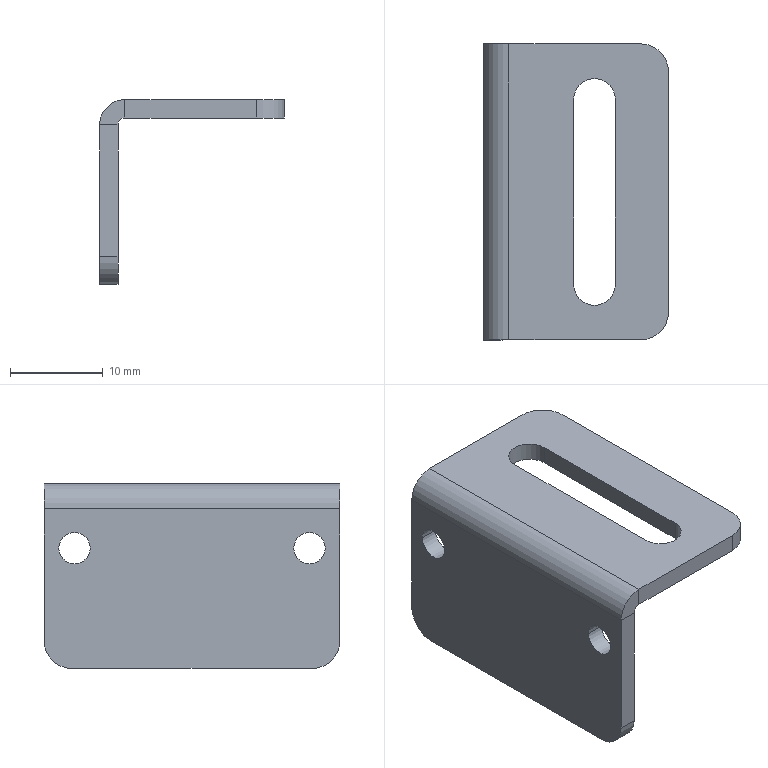Component | SolidWorks | 09-1111-12 | 1 solid | 26 faces | box 20 x 32 x 20 mm | volume 2121 mm3 | plane 14 | cylinder 12 | commonest cylinder face diameters 3.4 x4 6 x4 4.5 x2 5.473 x1 1.473 x1
STEP:
#1=COLOUR_RGB('',0.7922,0.8196,0.9333);
#2=FILL_AREA_STYLE_COLOUR('',#1);
#3=FILL_AREA_STYLE('',(#2));
#4=SURFACE_STYLE_FILL_AREA(#3);
#5=SURFACE_SIDE_STYLE('',(#4));
#6=SURFACE_STYLE_USAGE(.BOTH.,#5);
#7=PRESENTATION_STYLE_ASSIGNMENT((#6));
#8=CARTESIAN_POINT('',(5.115,16.78,49.727));
#9=VERTEX_POINT('',#8);
#10=CARTESIAN_POINT('',(5.115,16.914,49.727));
#11=VERTEX_POINT('',#10);
#12=CARTESIAN_POINT('',(5.115,16.847,49.727));
#13=DIRECTION('',(-1.,-0.,0.));
#14=DIRECTION('',(0.,1.,0.));
#15=AXIS2_PLACEMENT_3D('',#12,#13,#14);
#16=CIRCLE('',#15,0.06693);
#17=EDGE_CURVE('',#9,#11,#16,.T.);
#18=ORIENTED_EDGE('',*,*,#17,.F.);
#19=CARTESIAN_POINT('',(5.037,16.78,49.727));
#20=VERTEX_POINT('',#19);
#21=CARTESIAN_POINT('',(5.037,16.78,49.727));
#22=DIRECTION('',(-1.,-0.,0.));
#23=VECTOR('',#22,39.37);
#24=LINE('',#21,#23);
#25=EDGE_CURVE('',#9,#20,#24,.T.);
#26=ORIENTED_EDGE('',*,*,#25,.T.);
#27=CARTESIAN_POINT('',(5.037,16.914,49.727));
#28=VERTEX_POINT('',#27);
#29=CARTESIAN_POINT('',(5.037,16.847,49.727));
#30=DIRECTION('',(-1.,-0.,0.));
#31=DIRECTION('',(0.,1.,0.));
#32=AXIS2_PLACEMENT_3D('',#29,#30,#31);
#33=CIRCLE('',#32,0.06693);
#34=EDGE_CURVE('',#20,#28,#33,.T.);
#35=ORIENTED_EDGE('',*,*,#34,.T.);
#36=CARTESIAN_POINT('',(5.037,16.914,49.727));
#37=DIRECTION('',(-1.,-0.,0.));
#38=VECTOR('',#37,39.37);
#39=LINE('',#36,#38);
#40=EDGE_CURVE('',#11,#28,#39,.T.);
#41=ORIENTED_EDGE('',*,*,#40,.F.);
#42=EDGE_LOOP('',(#18,#26,#35,#41));
#43=FACE_OUTER_BOUND('',#42,.T.);
#44=CARTESIAN_POINT('',(5.037,16.847,49.727));
#45=DIRECTION('',(-1.,-0.,0.));
#46=DIRECTION('',(0.,1.,0.));
#47=AXIS2_PLACEMENT_3D('',#44,#45,#46);
#48=CYLINDRICAL_SURFACE('',#47,0.06693);
#49=ADVANCED_FACE('',(#43),#48,.F.);
#50=CARTESIAN_POINT('',(5.115,15.78,49.727));
#51=VERTEX_POINT('',#50);
#52=CARTESIAN_POINT('',(5.115,15.914,49.727));
#53=VERTEX_POINT('',#52);
#54=CARTESIAN_POINT('',(5.115,15.847,49.727));
#55=DIRECTION('',(-1.,-0.,0.));
#56=DIRECTION('',(0.,1.,0.));
#57=AXIS2_PLACEMENT_3D('',#54,#55,#56);
#58=CIRCLE('',#57,0.06693);
#59=EDGE_CURVE('',#51,#53,#58,.T.);
#60=ORIENTED_EDGE('',*,*,#59,.F.);
#61=CARTESIAN_POINT('',(5.037,15.78,49.727));
#62=VERTEX_POINT('',#61);
#63=CARTESIAN_POINT('',(5.037,15.78,49.727));
#64=DIRECTION('',(-1.,-0.,0.));
#65=VECTOR('',#64,39.37);
#66=LINE('',#63,#65);
#67=EDGE_CURVE('',#51,#62,#66,.T.);
#68=ORIENTED_EDGE('',*,*,#67,.T.);
#69=CARTESIAN_POINT('',(5.037,15.914,49.727));
#70=VERTEX_POINT('',#69);
#71=CARTESIAN_POINT('',(5.037,15.847,49.727));
#72=DIRECTION('',(-1.,-0.,0.));
#73=DIRECTION('',(0.,1.,0.));
#74=AXIS2_PLACEMENT_3D('',#71,#72,#73);
#75=CIRCLE('',#74,0.06693);
#76=EDGE_CURVE('',#62,#70,#75,.T.);
#77=ORIENTED_EDGE('',*,*,#76,.T.);
#78=CARTESIAN_POINT('',(5.037,15.914,49.727));
#79=DIRECTION('',(-1.,-0.,0.));
#80=VECTOR('',#79,39.37);
#81=LINE('',#78,#80);
#82=EDGE_CURVE('',#53,#70,#81,.T.);
#83=ORIENTED_EDGE('',*,*,#82,.F.);
#84=EDGE_LOOP('',(#60,#68,#77,#83));
#85=FACE_OUTER_BOUND('',#84,.T.);
#86=CARTESIAN_POINT('',(5.037,15.847,49.727));
#87=DIRECTION('',(-1.,-0.,0.));
#88=DIRECTION('',(0.,1.,0.));
#89=AXIS2_PLACEMENT_3D('',#86,#87,#88);
#90=CYLINDRICAL_SURFACE('',#89,0.06693);
#91=ADVANCED_FACE('',(#85),#90,.F.);
#92=CARTESIAN_POINT('',(5.037,16.977,49.894));
#93=VERTEX_POINT('',#92);
#94=CARTESIAN_POINT('',(5.115,16.977,49.894));
#95=VERTEX_POINT('',#94);
#96=CARTESIAN_POINT('',(5.037,16.977,49.894));
#97=DIRECTION('',(1.,0.,-0.));
#98=VECTOR('',#97,39.37);
#99=LINE('',#96,#98);
#100=EDGE_CURVE('',#93,#95,#99,.T.);
#101=ORIENTED_EDGE('',*,*,#100,.F.);
#102=CARTESIAN_POINT('',(5.144,16.977,50.002));
#103=VERTEX_POINT('',#102);
#104=CARTESIAN_POINT('',(5.144,16.977,49.894));
#105=DIRECTION('',(0.,-1.,0.));
#106=DIRECTION('',(1.,0.,0.));
#107=AXIS2_PLACEMENT_3D('',#104,#105,#106);
#108=CIRCLE('',#107,0.1077);
#109=EDGE_CURVE('',#103,#93,#108,.T.);
#110=ORIENTED_EDGE('',*,*,#109,.F.);
#111=CARTESIAN_POINT('',(5.144,16.977,49.923));
#112=VERTEX_POINT('',#111);
#113=CARTESIAN_POINT('',(5.144,16.977,49.923));
#114=DIRECTION('',(0.,0.,1.));
#115=VECTOR('',#114,39.37);
#116=LINE('',#113,#115);
#117=EDGE_CURVE('',#112,#103,#116,.T.);
#118=ORIENTED_EDGE('',*,*,#117,.F.);
#119=CARTESIAN_POINT('',(5.144,16.977,49.894));
#120=DIRECTION('',(0.,-1.,0.));
#121=DIRECTION('',(1.,0.,0.));
#122=AXIS2_PLACEMENT_3D('',#119,#120,#121);
#123=CIRCLE('',#122,0.029);
#124=EDGE_CURVE('',#112,#95,#123,.T.);
#125=ORIENTED_EDGE('',*,*,#124,.T.);
#126=EDGE_LOOP('',(#101,#110,#118,#125));
#127=FACE_OUTER_BOUND('',#126,.T.);
#128=CARTESIAN_POINT('',(5.037,16.977,49.894));
#129=DIRECTION('',(-0.,1.,-0.));
#130=DIRECTION('',(1.,0.,-0.));
#131=AXIS2_PLACEMENT_3D('',#128,#129,#130);
#132=PLANE('',#131);
#133=ADVANCED_FACE('',(#127),#132,.T.);
#134=CARTESIAN_POINT('',(5.115,16.977,49.333));
#135=VERTEX_POINT('',#134);
#136=CARTESIAN_POINT('',(5.115,16.977,50.002));
#137=DIRECTION('',(-0.,-0.,-1.));
#138=VECTOR('',#137,39.37);
#139=LINE('',#136,#138);
#140=EDGE_CURVE('',#95,#135,#139,.T.);
#141=ORIENTED_EDGE('',*,*,#140,.T.);
#142=CARTESIAN_POINT('',(5.037,16.977,49.333));
#143=VERTEX_POINT('',#142);
#144=CARTESIAN_POINT('',(5.144,16.977,49.333));
#145=DIRECTION('',(-1.,-0.,0.));
#146=VECTOR('',#145,39.37);
#147=LINE('',#144,#146);
#148=EDGE_CURVE('',#135,#143,#147,.T.);
#149=ORIENTED_EDGE('',*,*,#148,.T.);
#150=CARTESIAN_POINT('',(5.037,16.977,50.002));
#151=DIRECTION('',(-0.,-0.,-1.));
#152=VECTOR('',#151,39.37);
#153=LINE('',#150,#152);
#154=EDGE_CURVE('',#93,#143,#153,.T.);
#155=ORIENTED_EDGE('',*,*,#154,.F.);
#156=ORIENTED_EDGE('',*,*,#100,.T.);
#157=EDGE_LOOP('',(#141,#149,#155,#156));
#158=FACE_OUTER_BOUND('',#157,.T.);
#159=CARTESIAN_POINT('',(5.144,16.977,49.923));
#160=DIRECTION('',(-0.,1.,-0.));
#161=DIRECTION('',(1.,0.,-0.));
#162=AXIS2_PLACEMENT_3D('',#159,#160,#161);
#163=PLANE('',#162);
#164=ADVANCED_FACE('',(#158),#163,.T.);
#165=CARTESIAN_POINT('',(5.144,15.717,50.002));
#166=VERTEX_POINT('',#165);
#167=CARTESIAN_POINT('',(5.144,15.717,49.923));
#168=VERTEX_POINT('',#167);
#169=CARTESIAN_POINT('',(5.144,15.717,50.002));
#170=DIRECTION('',(-0.,-0.,-1.));
#171=VECTOR('',#170,39.37);
#172=LINE('',#169,#171);
#173=EDGE_CURVE('',#166,#168,#172,.T.);
#174=ORIENTED_EDGE('',*,*,#173,.F.);
#175=CARTESIAN_POINT('',(5.037,15.717,49.894));
#176=VERTEX_POINT('',#175);
#177=CARTESIAN_POINT('',(5.144,15.717,49.894));
#178=DIRECTION('',(0.,-1.,0.));
#179=DIRECTION('',(1.,0.,0.));
#180=AXIS2_PLACEMENT_3D('',#177,#178,#179);
#181=CIRCLE('',#180,0.1077);
#182=EDGE_CURVE('',#166,#176,#181,.T.);
#183=ORIENTED_EDGE('',*,*,#182,.T.);
#184=CARTESIAN_POINT('',(5.115,15.717,49.894));
#185=VERTEX_POINT('',#184);
#186=CARTESIAN_POINT('',(5.115,15.717,49.894));
#187=DIRECTION('',(-1.,-0.,0.));
#188=VECTOR('',#187,39.37);
#189=LINE('',#186,#188);
#190=EDGE_CURVE('',#185,#176,#189,.T.);
#191=ORIENTED_EDGE('',*,*,#190,.F.);
#192=CARTESIAN_POINT('',(5.144,15.717,49.894));
#193=DIRECTION('',(0.,-1.,0.));
#194=DIRECTION('',(1.,0.,0.));
#195=AXIS2_PLACEMENT_3D('',#192,#193,#194);
#196=CIRCLE('',#195,0.029);
#197=EDGE_CURVE('',#168,#185,#196,.T.);
#198=ORIENTED_EDGE('',*,*,#197,.F.);
#199=EDGE_LOOP('',(#174,#183,#191,#198));
#200=FACE_OUTER_BOUND('',#199,.T.);
#201=CARTESIAN_POINT('',(5.144,15.717,50.002));
#202=DIRECTION('',(0.,-1.,0.));
#203=DIRECTION('',(-1.,-0.,0.));
#204=AXIS2_PLACEMENT_3D('',#201,#202,#203);
#205=PLANE('',#204);
#206=ADVANCED_FACE('',(#200),#205,.T.);
#207=CARTESIAN_POINT('',(5.706,15.717,49.923));
#208=VERTEX_POINT('',#207);
#209=CARTESIAN_POINT('',(5.824,15.717,49.923));
#210=DIRECTION('',(-1.,-0.,0.));
#211=VECTOR('',#210,39.37);
#212=LINE('',#209,#211);
#213=EDGE_CURVE('',#208,#168,#212,.T.);
#214=ORIENTED_EDGE('',*,*,#213,.F.);
#215=CARTESIAN_POINT('',(5.706,15.717,50.002));
#216=VERTEX_POINT('',#215);
#217=CARTESIAN_POINT('',(5.706,15.717,49.894));
#218=DIRECTION('',(0.,0.,1.));
#219=VECTOR('',#218,39.37);
#220=LINE('',#217,#219);
#221=EDGE_CURVE('',#208,#216,#220,.T.);
#222=ORIENTED_EDGE('',*,*,#221,.T.);
#223=CARTESIAN_POINT('',(5.824,15.717,50.002));
#224=DIRECTION('',(-1.,-0.,0.));
#225=VECTOR('',#224,39.37);
#226=LINE('',#223,#225);
#227=EDGE_CURVE('',#216,#166,#226,.T.);
#228=ORIENTED_EDGE('',*,*,#227,.T.);
#229=ORIENTED_EDGE('',*,*,#173,.T.);
#230=EDGE_LOOP('',(#214,#222,#228,#229));
#231=FACE_OUTER_BOUND('',#230,.T.);
#232=CARTESIAN_POINT('',(5.115,15.717,49.894));
#233=DIRECTION('',(0.,-1.,0.));
#234=DIRECTION('',(-1.,-0.,0.));
#235=AXIS2_PLACEMENT_3D('',#232,#233,#234);
#236=PLANE('',#235);
#237=ADVANCED_FACE('',(#231),#236,.T.);
#238=CARTESIAN_POINT('',(5.115,16.847,49.727));
#239=DIRECTION('',(-1.,-0.,0.));
#240=DIRECTION('',(0.,1.,0.));
#241=AXIS2_PLACEMENT_3D('',#238,#239,#240);
#242=CIRCLE('',#241,0.06693);
#243=EDGE_CURVE('',#11,#9,#242,.T.);
#244=ORIENTED_EDGE('',*,*,#243,.T.);
#245=ORIENTED_EDGE('',*,*,#17,.T.);
#246=EDGE_LOOP('',(#244,#245));
#247=FACE_BOUND('',#246,.T.);
#248=CARTESIAN_POINT('',(5.115,15.847,49.727));
#249=DIRECTION('',(-1.,-0.,0.));
#250=DIRECTION('',(0.,1.,0.));
#251=AXIS2_PLACEMENT_3D('',#248,#249,#250);
#252=CIRCLE('',#251,0.06693);
#253=EDGE_CURVE('',#53,#51,#252,.T.);
#254=ORIENTED_EDGE('',*,*,#253,.T.);
#255=ORIENTED_EDGE('',*,*,#59,.T.);
#256=EDGE_LOOP('',(#254,#255));
#257=FACE_BOUND('',#256,.T.);
#258=CARTESIAN_POINT('',(5.115,16.859,49.215));
#259=VERTEX_POINT('',#258);
#260=CARTESIAN_POINT('',(5.115,15.836,49.215));
#261=VERTEX_POINT('',#260);
#262=CARTESIAN_POINT('',(5.115,16.977,49.215));
#263=DIRECTION('',(0.,-1.,0.));
#264=VECTOR('',#263,39.37);
#265=LINE('',#262,#264);
#266=EDGE_CURVE('',#259,#261,#265,.T.);
#267=ORIENTED_EDGE('',*,*,#266,.F.);
#268=CARTESIAN_POINT('',(5.115,16.859,49.333));
#269=DIRECTION('',(1.,0.,-0.));
#270=DIRECTION('',(0.,1.,0.));
#271=AXIS2_PLACEMENT_3D('',#268,#269,#270);
#272=CIRCLE('',#271,0.1181);
#273=EDGE_CURVE('',#259,#135,#272,.T.);
#274=ORIENTED_EDGE('',*,*,#273,.T.);
#275=ORIENTED_EDGE('',*,*,#140,.F.);
#276=CARTESIAN_POINT('',(5.115,16.977,49.894));
#277=DIRECTION('',(0.,-1.,0.));
#278=VECTOR('',#277,39.37);
#279=LINE('',#276,#278);
#280=EDGE_CURVE('',#95,#185,#279,.T.);
#281=ORIENTED_EDGE('',*,*,#280,.T.);
#282=CARTESIAN_POINT('',(5.115,15.717,49.333));
#283=VERTEX_POINT('',#282);
#284=CARTESIAN_POINT('',(5.115,15.717,50.002));
#285=DIRECTION('',(-0.,-0.,-1.));
#286=VECTOR('',#285,39.37);
#287=LINE('',#284,#286);
#288=EDGE_CURVE('',#185,#283,#287,.T.);
#289=ORIENTED_EDGE('',*,*,#288,.T.);
#290=CARTESIAN_POINT('',(5.115,15.836,49.333));
#291=DIRECTION('',(1.,0.,-0.));
#292=DIRECTION('',(0.,1.,0.));
#293=AXIS2_PLACEMENT_3D('',#290,#291,#292);
#294=CIRCLE('',#293,0.1181);
#295=EDGE_CURVE('',#283,#261,#294,.T.);
#296=ORIENTED_EDGE('',*,*,#295,.T.);
#297=EDGE_LOOP('',(#267,#274,#275,#281,#289,#296));
#298=FACE_OUTER_BOUND('',#297,.T.);
#299=CARTESIAN_POINT('',(5.115,16.977,50.002));
#300=DIRECTION('',(-1.,-0.,0.));
#301=DIRECTION('',(-0.,1.,-0.));
#302=AXIS2_PLACEMENT_3D('',#299,#300,#301);
#303=PLANE('',#302);
#304=ADVANCED_FACE('',(#247,#257,#298),#303,.F.);
#305=CARTESIAN_POINT('',(5.037,16.859,49.215));
#306=VERTEX_POINT('',#305);
#307=CARTESIAN_POINT('',(5.037,15.836,49.215));
#308=VERTEX_POINT('',#307);
#309=CARTESIAN_POINT('',(5.037,16.977,49.215));
#310=DIRECTION('',(0.,-1.,0.));
#311=VECTOR('',#310,39.37);
#312=LINE('',#309,#311);
#313=EDGE_CURVE('',#306,#308,#312,.T.);
#314=ORIENTED_EDGE('',*,*,#313,.F.);
#315=CARTESIAN_POINT('',(5.037,16.859,49.215));
#316=DIRECTION('',(1.,0.,-0.));
#317=VECTOR('',#316,39.37);
#318=LINE('',#315,#317);
#319=EDGE_CURVE('',#306,#259,#318,.T.);
#320=ORIENTED_EDGE('',*,*,#319,.T.);
#321=ORIENTED_EDGE('',*,*,#266,.T.);
#322=CARTESIAN_POINT('',(5.037,15.836,49.215));
#323=DIRECTION('',(-1.,-0.,0.));
#324=VECTOR('',#323,39.37);
#325=LINE('',#322,#324);
#326=EDGE_CURVE('',#261,#308,#325,.T.);
#327=ORIENTED_EDGE('',*,*,#326,.T.);
#328=EDGE_LOOP('',(#314,#320,#321,#327));
#329=FACE_OUTER_BOUND('',#328,.T.);
#330=CARTESIAN_POINT('',(5.037,16.977,49.215));
#331=DIRECTION('',(-0.,-0.,-1.));
#332=DIRECTION('',(-0.,1.,-0.));
#333=AXIS2_PLACEMENT_3D('',#330,#331,#332);
#334=PLANE('',#333);
#335=ADVANCED_FACE('',(#329),#334,.T.);
#336=CARTESIAN_POINT('',(5.037,16.847,49.727));
#337=DIRECTION('',(-1.,-0.,0.));
#338=DIRECTION('',(0.,1.,0.));
#339=AXIS2_PLACEMENT_3D('',#336,#337,#338);
#340=CIRCLE('',#339,0.06693);
#341=EDGE_CURVE('',#28,#20,#340,.T.);
#342=ORIENTED_EDGE('',*,*,#341,.F.);
#343=ORIENTED_EDGE('',*,*,#34,.F.);
#344=EDGE_LOOP('',(#342,#343));
#345=FACE_BOUND('',#344,.T.);
#346=CARTESIAN_POINT('',(5.037,15.847,49.727));
#347=DIRECTION('',(-1.,-0.,0.));
#348=DIRECTION('',(0.,1.,0.));
#349=AXIS2_PLACEMENT_3D('',#346,#347,#348);
#350=CIRCLE('',#349,0.06693);
#351=EDGE_CURVE('',#70,#62,#350,.T.);
#352=ORIENTED_EDGE('',*,*,#351,.F.);
#353=ORIENTED_EDGE('',*,*,#76,.F.);
#354=EDGE_LOOP('',(#352,#353));
#355=FACE_BOUND('',#354,.T.);
#356=ORIENTED_EDGE('',*,*,#154,.T.);
#357=CARTESIAN_POINT('',(5.037,16.859,49.333));
#358=DIRECTION('',(-1.,-0.,0.));
#359=DIRECTION('',(0.,1.,0.));
#360=AXIS2_PLACEMENT_3D('',#357,#358,#359);
#361=CIRCLE('',#360,0.1181);
#362=EDGE_CURVE('',#143,#306,#361,.T.);
#363=ORIENTED_EDGE('',*,*,#362,.T.);
#364=ORIENTED_EDGE('',*,*,#313,.T.);
#365=CARTESIAN_POINT('',(5.037,15.717,49.333));
#366=VERTEX_POINT('',#365);
#367=CARTESIAN_POINT('',(5.037,15.836,49.333));
#368=DIRECTION('',(-1.,-0.,0.));
#369=DIRECTION('',(0.,1.,0.));
#370=AXIS2_PLACEMENT_3D('',#367,#368,#369);
#371=CIRCLE('',#370,0.1181);
#372=EDGE_CURVE('',#308,#366,#371,.T.);
#373=ORIENTED_EDGE('',*,*,#372,.T.);
#374=CARTESIAN_POINT('',(5.037,15.717,50.002));
#375=DIRECTION('',(-0.,-0.,-1.));
#376=VECTOR('',#375,39.37);
#377=LINE('',#374,#376);
#378=EDGE_CURVE('',#176,#366,#377,.T.);
#379=ORIENTED_EDGE('',*,*,#378,.F.);
#380=CARTESIAN_POINT('',(5.037,16.977,49.894));
#381=DIRECTION('',(0.,-1.,0.));
#382=VECTOR('',#381,39.37);
#383=LINE('',#380,#382);
#384=EDGE_CURVE('',#93,#176,#383,.T.);
#385=ORIENTED_EDGE('',*,*,#384,.F.);
#386=EDGE_LOOP('',(#356,#363,#364,#373,#379,#385));
#387=FACE_OUTER_BOUND('',#386,.T.);
#388=CARTESIAN_POINT('',(5.037,16.977,50.002));
#389=DIRECTION('',(-1.,-0.,0.));
#390=DIRECTION('',(-0.,1.,-0.));
#391=AXIS2_PLACEMENT_3D('',#388,#389,#390);
#392=PLANE('',#391);
#393=ADVANCED_FACE('',(#345,#355,#387),#392,.T.);
#394=ORIENTED_EDGE('',*,*,#182,.F.);
#395=CARTESIAN_POINT('',(5.144,16.977,50.002));
#396=DIRECTION('',(0.,-1.,0.));
#397=VECTOR('',#396,39.37);
#398=LINE('',#395,#397);
#399=EDGE_CURVE('',#103,#166,#398,.T.);
#400=ORIENTED_EDGE('',*,*,#399,.F.);
#401=ORIENTED_EDGE('',*,*,#109,.T.);
#402=ORIENTED_EDGE('',*,*,#384,.T.);
#403=EDGE_LOOP('',(#394,#400,#401,#402));
#404=FACE_OUTER_BOUND('',#403,.T.);
#405=CARTESIAN_POINT('',(5.144,16.977,49.894));
#406=DIRECTION('',(0.,-1.,0.));
#407=DIRECTION('',(-1.,0.,0.));
#408=AXIS2_PLACEMENT_3D('',#405,#406,#407);
#409=CYLINDRICAL_SURFACE('',#408,0.1077);
#410=ADVANCED_FACE('',(#404),#409,.T.);
#411=CARTESIAN_POINT('',(5.42,16.741,50.002));
#412=VERTEX_POINT('',#411);
#413=CARTESIAN_POINT('',(5.598,16.741,50.002));
#414=VERTEX_POINT('',#413);
#415=CARTESIAN_POINT('',(5.509,16.741,50.002));
#416=DIRECTION('',(-0.,-0.,-1.));
#417=DIRECTION('',(-1.,0.,0.));
#418=AXIS2_PLACEMENT_3D('',#415,#416,#417);
#419=CIRCLE('',#418,0.08858);
#420=EDGE_CURVE('',#412,#414,#419,.T.);
#421=ORIENTED_EDGE('',*,*,#420,.T.);
#422=CARTESIAN_POINT('',(5.598,15.954,50.002));
#423=VERTEX_POINT('',#422);
#424=CARTESIAN_POINT('',(5.598,16.741,50.002));
#425=DIRECTION('',(0.,-1.,0.));
#426=VECTOR('',#425,39.37);
#427=LINE('',#424,#426);
#428=EDGE_CURVE('',#414,#423,#427,.T.);
#429=ORIENTED_EDGE('',*,*,#428,.T.);
#430=CARTESIAN_POINT('',(5.42,15.954,50.002));
#431=VERTEX_POINT('',#430);
#432=CARTESIAN_POINT('',(5.509,15.954,50.002));
#433=DIRECTION('',(-0.,-0.,-1.));
#434=DIRECTION('',(-1.,0.,0.));
#435=AXIS2_PLACEMENT_3D('',#432,#433,#434);
#436=CIRCLE('',#435,0.08858);
#437=EDGE_CURVE('',#423,#431,#436,.T.);
#438=ORIENTED_EDGE('',*,*,#437,.T.);
#439=CARTESIAN_POINT('',(5.42,16.741,50.002));
#440=DIRECTION('',(-0.,1.,-0.));
#441=VECTOR('',#440,39.37);
#442=LINE('',#439,#441);
#443=EDGE_CURVE('',#431,#412,#442,.T.);
#444=ORIENTED_EDGE('',*,*,#443,.T.);
#445=EDGE_LOOP('',(#421,#429,#438,#444));
#446=FACE_BOUND('',#445,.T.);
#447=ORIENTED_EDGE('',*,*,#227,.F.);
#448=CARTESIAN_POINT('',(5.824,15.836,50.002));
#449=VERTEX_POINT('',#448);
#450=CARTESIAN_POINT('',(5.706,15.836,50.002));
#451=DIRECTION('',(0.,0.,1.));
#452=DIRECTION('',(1.,0.,0.));
#453=AXIS2_PLACEMENT_3D('',#450,#451,#452);
#454=CIRCLE('',#453,0.1181);
#455=EDGE_CURVE('',#216,#449,#454,.T.);
#456=ORIENTED_EDGE('',*,*,#455,.T.);
#457=CARTESIAN_POINT('',(5.824,16.859,50.002));
#458=VERTEX_POINT('',#457);
#459=CARTESIAN_POINT('',(5.824,16.977,50.002));
#460=DIRECTION('',(0.,-1.,0.));
#461=VECTOR('',#460,39.37);
#462=LINE('',#459,#461);
#463=EDGE_CURVE('',#458,#449,#462,.T.);
#464=ORIENTED_EDGE('',*,*,#463,.F.);
#465=CARTESIAN_POINT('',(5.706,16.977,50.002));
#466=VERTEX_POINT('',#465);
#467=CARTESIAN_POINT('',(5.706,16.859,50.002));
#468=DIRECTION('',(0.,0.,1.));
#469=DIRECTION('',(1.,0.,0.));
#470=AXIS2_PLACEMENT_3D('',#467,#468,#469);
#471=CIRCLE('',#470,0.1181);
#472=EDGE_CURVE('',#458,#466,#471,.T.);
#473=ORIENTED_EDGE('',*,*,#472,.T.);
#474=CARTESIAN_POINT('',(5.824,16.977,50.002));
#475=DIRECTION('',(-1.,-0.,0.));
#476=VECTOR('',#475,39.37);
#477=LINE('',#474,#476);
#478=EDGE_CURVE('',#466,#103,#477,.T.);
#479=ORIENTED_EDGE('',*,*,#478,.T.);
#480=ORIENTED_EDGE('',*,*,#399,.T.);
#481=EDGE_LOOP('',(#447,#456,#464,#473,#479,#480));
#482=FACE_OUTER_BOUND('',#481,.T.);
#483=CARTESIAN_POINT('',(5.824,16.977,50.002));
#484=DIRECTION('',(0.,0.,1.));
#485=DIRECTION('',(1.,0.,-0.));
#486=AXIS2_PLACEMENT_3D('',#483,#484,#485);
#487=PLANE('',#486);
#488=ADVANCED_FACE('',(#446,#482),#487,.T.);
#489=ORIENTED_EDGE('',*,*,#463,.T.);
#490=CARTESIAN_POINT('',(5.824,15.836,49.923));
#491=VERTEX_POINT('',#490);
#492=CARTESIAN_POINT('',(5.824,15.836,49.923));
#493=DIRECTION('',(-0.,-0.,-1.));
#494=VECTOR('',#493,39.37);
#495=LINE('',#492,#494);
#496=EDGE_CURVE('',#449,#491,#495,.T.);
#497=ORIENTED_EDGE('',*,*,#496,.T.);
#498=CARTESIAN_POINT('',(5.824,16.859,49.923));
#499=VERTEX_POINT('',#498);
#500=CARTESIAN_POINT('',(5.824,16.977,49.923));
#501=DIRECTION('',(0.,-1.,0.));
#502=VECTOR('',#501,39.37);
#503=LINE('',#500,#502);
#504=EDGE_CURVE('',#499,#491,#503,.T.);
#505=ORIENTED_EDGE('',*,*,#504,.F.);
#506=CARTESIAN_POINT('',(5.824,16.859,49.923));
#507=DIRECTION('',(0.,0.,1.));
#508=VECTOR('',#507,39.37);
#509=LINE('',#506,#508);
#510=EDGE_CURVE('',#499,#458,#509,.T.);
#511=ORIENTED_EDGE('',*,*,#510,.T.);
#512=EDGE_LOOP('',(#489,#497,#505,#511));
#513=FACE_OUTER_BOUND('',#512,.T.);
#514=CARTESIAN_POINT('',(5.824,16.977,49.923));
#515=DIRECTION('',(1.,0.,-0.));
#516=DIRECTION('',(-0.,-0.,-1.));
#517=AXIS2_PLACEMENT_3D('',#514,#515,#516);
#518=PLANE('',#517);
#519=ADVANCED_FACE('',(#513),#518,.T.);
#520=CARTESIAN_POINT('',(5.598,16.741,49.923));
#521=VERTEX_POINT('',#520);
#522=CARTESIAN_POINT('',(5.598,15.954,49.923));
#523=VERTEX_POINT('',#522);
#524=CARTESIAN_POINT('',(5.598,16.741,49.923));
#525=DIRECTION('',(0.,-1.,0.));
#526=VECTOR('',#525,39.37);
#527=LINE('',#524,#526);
#528=EDGE_CURVE('',#521,#523,#527,.T.);
#529=ORIENTED_EDGE('',*,*,#528,.F.);
#530=CARTESIAN_POINT('',(5.42,16.741,49.923));
#531=VERTEX_POINT('',#530);
#532=CARTESIAN_POINT('',(5.509,16.741,49.923));
#533=DIRECTION('',(-0.,-0.,-1.));
#534=DIRECTION('',(-1.,0.,0.));
#535=AXIS2_PLACEMENT_3D('',#532,#533,#534);
#536=CIRCLE('',#535,0.08858);
#537=EDGE_CURVE('',#531,#521,#536,.T.);
#538=ORIENTED_EDGE('',*,*,#537,.F.);
#539=CARTESIAN_POINT('',(5.42,15.954,49.923));
#540=VERTEX_POINT('',#539);
#541=CARTESIAN_POINT('',(5.42,16.741,49.923));
#542=DIRECTION('',(-0.,1.,-0.));
#543=VECTOR('',#542,39.37);
#544=LINE('',#541,#543);
#545=EDGE_CURVE('',#540,#531,#544,.T.);
#546=ORIENTED_EDGE('',*,*,#545,.F.);
#547=CARTESIAN_POINT('',(5.509,15.954,49.923));
#548=DIRECTION('',(-0.,-0.,-1.));
#549=DIRECTION('',(-1.,0.,0.));
#550=AXIS2_PLACEMENT_3D('',#547,#548,#549);
#551=CIRCLE('',#550,0.08858);
#552=EDGE_CURVE('',#523,#540,#551,.T.);
#553=ORIENTED_EDGE('',*,*,#552,.F.);
#554=EDGE_LOOP('',(#529,#538,#546,#553));
#555=FACE_BOUND('',#554,.T.);
#556=ORIENTED_EDGE('',*,*,#504,.T.);
#557=CARTESIAN_POINT('',(5.706,15.836,49.923));
#558=DIRECTION('',(-0.,-0.,-1.));
#559=DIRECTION('',(1.,0.,0.));
#560=AXIS2_PLACEMENT_3D('',#557,#558,#559);
#561=CIRCLE('',#560,0.1181);
#562=EDGE_CURVE('',#491,#208,#561,.T.);
#563=ORIENTED_EDGE('',*,*,#562,.T.);
#564=ORIENTED_EDGE('',*,*,#213,.T.);
#565=CARTESIAN_POINT('',(5.144,16.977,49.923));
#566=DIRECTION('',(0.,-1.,0.));
#567=VECTOR('',#566,39.37);
#568=LINE('',#565,#567);
#569=EDGE_CURVE('',#112,#168,#568,.T.);
#570=ORIENTED_EDGE('',*,*,#569,.F.);
#571=CARTESIAN_POINT('',(5.706,16.977,49.923));
#572=VERTEX_POINT('',#571);
#573=CARTESIAN_POINT('',(5.824,16.977,49.923));
#574=DIRECTION('',(-1.,-0.,0.));
#575=VECTOR('',#574,39.37);
#576=LINE('',#573,#575);
#577=EDGE_CURVE('',#572,#112,#576,.T.);
#578=ORIENTED_EDGE('',*,*,#577,.F.);
#579=CARTESIAN_POINT('',(5.706,16.859,49.923));
#580=DIRECTION('',(-0.,-0.,-1.));
#581=DIRECTION('',(1.,0.,0.));
#582=AXIS2_PLACEMENT_3D('',#579,#580,#581);
#583=CIRCLE('',#582,0.1181);
#584=EDGE_CURVE('',#572,#499,#583,.T.);
#585=ORIENTED_EDGE('',*,*,#584,.T.);
#586=EDGE_LOOP('',(#556,#563,#564,#570,#578,#585));
#587=FACE_OUTER_BOUND('',#586,.T.);
#588=CARTESIAN_POINT('',(5.824,16.977,49.923));
#589=DIRECTION('',(0.,0.,1.));
#590=DIRECTION('',(1.,0.,-0.));
#591=AXIS2_PLACEMENT_3D('',#588,#589,#590);
#592=PLANE('',#591);
#593=ADVANCED_FACE('',(#555,#587),#592,.F.);
#594=ORIENTED_EDGE('',*,*,#197,.T.);
#595=ORIENTED_EDGE('',*,*,#280,.F.);
#596=ORIENTED_EDGE('',*,*,#124,.F.);
#597=ORIENTED_EDGE('',*,*,#569,.T.);
#598=EDGE_LOOP('',(#594,#595,#596,#597));
#599=FACE_OUTER_BOUND('',#598,.T.);
#600=CARTESIAN_POINT('',(5.144,16.977,49.894));
#601=DIRECTION('',(0.,-1.,0.));
#602=DIRECTION('',(-1.,0.,0.));
#603=AXIS2_PLACEMENT_3D('',#600,#601,#602);
#604=CYLINDRICAL_SURFACE('',#603,0.029);
#605=ADVANCED_FACE('',(#599),#604,.F.);
#606=ORIENTED_EDGE('',*,*,#478,.F.);
#607=CARTESIAN_POINT('',(5.706,16.977,49.894));
#608=DIRECTION('',(-0.,-0.,-1.));
#609=VECTOR('',#608,39.37);
#610=LINE('',#607,#609);
#611=EDGE_CURVE('',#466,#572,#610,.T.);
#612=ORIENTED_EDGE('',*,*,#611,.T.);
#613=ORIENTED_EDGE('',*,*,#577,.T.);
#614=ORIENTED_EDGE('',*,*,#117,.T.);
#615=EDGE_LOOP('',(#606,#612,#613,#614));
#616=FACE_OUTER_BOUND('',#615,.T.);
#617=CARTESIAN_POINT('',(5.144,16.977,49.894));
#618=DIRECTION('',(-0.,1.,-0.));
#619=DIRECTION('',(1.,0.,-0.));
#620=AXIS2_PLACEMENT_3D('',#617,#618,#619);
#621=PLANE('',#620);
#622=ADVANCED_FACE('',(#616),#621,.T.);
#623=ORIENTED_EDGE('',*,*,#378,.T.);
#624=CARTESIAN_POINT('',(5.115,15.717,49.333));
#625=DIRECTION('',(1.,0.,-0.));
#626=VECTOR('',#625,39.37);
#627=LINE('',#624,#626);
#628=EDGE_CURVE('',#366,#283,#627,.T.);
#629=ORIENTED_EDGE('',*,*,#628,.T.);
#630=ORIENTED_EDGE('',*,*,#288,.F.);
#631=ORIENTED_EDGE('',*,*,#190,.T.);
#632=EDGE_LOOP('',(#623,#629,#630,#631));
#633=FACE_OUTER_BOUND('',#632,.T.);
#634=CARTESIAN_POINT('',(5.144,15.717,49.894));
#635=DIRECTION('',(-0.,1.,-0.));
#636=DIRECTION('',(1.,0.,-0.));
#637=AXIS2_PLACEMENT_3D('',#634,#635,#636);
#638=PLANE('',#637);
#639=ADVANCED_FACE('',(#633),#638,.F.);
#640=ORIENTED_EDGE('',*,*,#67,.F.);
#641=ORIENTED_EDGE('',*,*,#253,.F.);
#642=ORIENTED_EDGE('',*,*,#82,.T.);
#643=ORIENTED_EDGE('',*,*,#351,.T.);
#644=EDGE_LOOP('',(#640,#641,#642,#643));
#645=FACE_OUTER_BOUND('',#644,.T.);
#646=CARTESIAN_POINT('',(5.037,15.847,49.727));
#647=DIRECTION('',(-1.,-0.,0.));
#648=DIRECTION('',(0.,1.,0.));
#649=AXIS2_PLACEMENT_3D('',#646,#647,#648);
#650=CYLINDRICAL_SURFACE('',#649,0.06693);
#651=ADVANCED_FACE('',(#645),#650,.F.);
#652=ORIENTED_EDGE('',*,*,#25,.F.);
#653=ORIENTED_EDGE('',*,*,#243,.F.);
#654=ORIENTED_EDGE('',*,*,#40,.T.);
#655=ORIENTED_EDGE('',*,*,#341,.T.);
#656=EDGE_LOOP('',(#652,#653,#654,#655));
#657=FACE_OUTER_BOUND('',#656,.T.);
#658=CARTESIAN_POINT('',(5.037,16.847,49.727));
#659=DIRECTION('',(-1.,-0.,0.));
#660=DIRECTION('',(0.,1.,0.));
#661=AXIS2_PLACEMENT_3D('',#658,#659,#660);
#662=CYLINDRICAL_SURFACE('',#661,0.06693);
#663=ADVANCED_FACE('',(#657),#662,.F.);
#664=ORIENTED_EDGE('',*,*,#537,.T.);
#665=CARTESIAN_POINT('',(5.598,16.741,50.002));
#666=DIRECTION('',(-0.,-0.,-1.));
#667=VECTOR('',#666,39.37);
#668=LINE('',#665,#667);
#669=EDGE_CURVE('',#414,#521,#668,.T.);
#670=ORIENTED_EDGE('',*,*,#669,.F.);
#671=ORIENTED_EDGE('',*,*,#420,.F.);
#672=CARTESIAN_POINT('',(5.42,16.741,50.002));
#673=DIRECTION('',(-0.,-0.,-1.));
#674=VECTOR('',#673,39.37);
#675=LINE('',#672,#674);
#676=EDGE_CURVE('',#412,#531,#675,.T.);
#677=ORIENTED_EDGE('',*,*,#676,.T.);
#678=EDGE_LOOP('',(#664,#670,#671,#677));
#679=FACE_OUTER_BOUND('',#678,.T.);
#680=CARTESIAN_POINT('',(5.509,16.741,50.002));
#681=DIRECTION('',(-0.,-0.,-1.));
#682=DIRECTION('',(-1.,0.,0.));
#683=AXIS2_PLACEMENT_3D('',#680,#681,#682);
#684=CYLINDRICAL_SURFACE('',#683,0.08858);
#685=ADVANCED_FACE('',(#679),#684,.F.);
#686=ORIENTED_EDGE('',*,*,#545,.T.);
#687=ORIENTED_EDGE('',*,*,#676,.F.);
#688=ORIENTED_EDGE('',*,*,#443,.F.);
#689=CARTESIAN_POINT('',(5.42,15.954,50.002));
#690=DIRECTION('',(-0.,-0.,-1.));
#691=VECTOR('',#690,39.37);
#692=LINE('',#689,#691);
#693=EDGE_CURVE('',#431,#540,#692,.T.);
#694=ORIENTED_EDGE('',*,*,#693,.T.);
#695=EDGE_LOOP('',(#686,#687,#688,#694));
#696=FACE_OUTER_BOUND('',#695,.T.);
#697=CARTESIAN_POINT('',(5.42,16.741,50.002));
#698=DIRECTION('',(-1.,-0.,0.));
#699=DIRECTION('',(0.,0.,1.));
#700=AXIS2_PLACEMENT_3D('',#697,#698,#699);
#701=PLANE('',#700);
#702=ADVANCED_FACE('',(#696),#701,.F.);
#703=ORIENTED_EDGE('',*,*,#552,.T.);
#704=ORIENTED_EDGE('',*,*,#693,.F.);
#705=ORIENTED_EDGE('',*,*,#437,.F.);
#706=CARTESIAN_POINT('',(5.598,15.954,50.002));
#707=DIRECTION('',(-0.,-0.,-1.));
#708=VECTOR('',#707,39.37);
#709=LINE('',#706,#708);
#710=EDGE_CURVE('',#423,#523,#709,.T.);
#711=ORIENTED_EDGE('',*,*,#710,.T.);
#712=EDGE_LOOP('',(#703,#704,#705,#711));
#713=FACE_OUTER_BOUND('',#712,.T.);
#714=CARTESIAN_POINT('',(5.509,15.954,50.002));
#715=DIRECTION('',(-0.,-0.,-1.));
#716=DIRECTION('',(-1.,0.,0.));
#717=AXIS2_PLACEMENT_3D('',#714,#715,#716);
#718=CYLINDRICAL_SURFACE('',#717,0.08858);
#719=ADVANCED_FACE('',(#713),#718,.F.);
#720=ORIENTED_EDGE('',*,*,#528,.T.);
#721=ORIENTED_EDGE('',*,*,#710,.F.);
#722=ORIENTED_EDGE('',*,*,#428,.F.);
#723=ORIENTED_EDGE('',*,*,#669,.T.);
#724=EDGE_LOOP('',(#720,#721,#722,#723));
#725=FACE_OUTER_BOUND('',#724,.T.);
#726=CARTESIAN_POINT('',(5.598,16.741,50.002));
#727=DIRECTION('',(1.,0.,-0.));
#728=DIRECTION('',(-0.,-0.,-1.));
#729=AXIS2_PLACEMENT_3D('',#726,#727,#728);
#730=PLANE('',#729);
#731=ADVANCED_FACE('',(#725),#730,.F.);
#732=ORIENTED_EDGE('',*,*,#562,.F.);
#733=ORIENTED_EDGE('',*,*,#496,.F.);
#734=ORIENTED_EDGE('',*,*,#455,.F.);
#735=ORIENTED_EDGE('',*,*,#221,.F.);
#736=EDGE_LOOP('',(#732,#733,#734,#735));
#737=FACE_OUTER_BOUND('',#736,.T.);
#738=CARTESIAN_POINT('',(5.706,15.836,49.894));
#739=DIRECTION('',(0.,0.,1.));
#740=DIRECTION('',(1.,0.,0.));
#741=AXIS2_PLACEMENT_3D('',#738,#739,#740);
#742=CYLINDRICAL_SURFACE('',#741,0.1181);
#743=ADVANCED_FACE('',(#737),#742,.T.);
#744=ORIENTED_EDGE('',*,*,#584,.F.);
#745=ORIENTED_EDGE('',*,*,#611,.F.);
#746=ORIENTED_EDGE('',*,*,#472,.F.);
#747=ORIENTED_EDGE('',*,*,#510,.F.);
#748=EDGE_LOOP('',(#744,#745,#746,#747));
#749=FACE_OUTER_BOUND('',#748,.T.);
#750=CARTESIAN_POINT('',(5.706,16.859,49.923));
#751=DIRECTION('',(0.,0.,1.));
#752=DIRECTION('',(1.,0.,0.));
#753=AXIS2_PLACEMENT_3D('',#750,#751,#752);
#754=CYLINDRICAL_SURFACE('',#753,0.1181);
#755=ADVANCED_FACE('',(#749),#754,.T.);
#756=ORIENTED_EDGE('',*,*,#362,.F.);
#757=ORIENTED_EDGE('',*,*,#148,.F.);
#758=ORIENTED_EDGE('',*,*,#273,.F.);
#759=ORIENTED_EDGE('',*,*,#319,.F.);
#760=EDGE_LOOP('',(#756,#757,#758,#759));
#761=FACE_OUTER_BOUND('',#760,.T.);
#762=CARTESIAN_POINT('',(5.037,16.859,49.333));
#763=DIRECTION('',(1.,0.,-0.));
#764=DIRECTION('',(0.,-1.,0.));
#765=AXIS2_PLACEMENT_3D('',#762,#763,#764);
#766=CYLINDRICAL_SURFACE('',#765,0.1181);
#767=ADVANCED_FACE('',(#761),#766,.T.);
#768=ORIENTED_EDGE('',*,*,#372,.F.);
#769=ORIENTED_EDGE('',*,*,#326,.F.);
#770=ORIENTED_EDGE('',*,*,#295,.F.);
#771=ORIENTED_EDGE('',*,*,#628,.F.);
#772=EDGE_LOOP('',(#768,#769,#770,#771));
#773=FACE_OUTER_BOUND('',#772,.T.);
#774=CARTESIAN_POINT('',(5.144,15.836,49.333));
#775=DIRECTION('',(-1.,-0.,0.));
#776=DIRECTION('',(0.,1.,0.));
#777=AXIS2_PLACEMENT_3D('',#774,#775,#776);
#778=CYLINDRICAL_SURFACE('',#777,0.1181);
#779=ADVANCED_FACE('',(#773),#778,.T.);
#780=CLOSED_SHELL('',(#49,#91,#133,#164,#206,#237,#304,#335,#393,#410,#488,#519,#593,#605,#622,#639,#651,#663,#685,#702,#719,#731,#743,#755,#767,#779));
#781=MANIFOLD_SOLID_BREP('',#780);
#782=STYLED_ITEM('',(#7),#781);
#783=PRESENTATION_LAYER_ASSIGNMENT('','',(#782));
#784=CARTESIAN_POINT('',(0.,0.,0.));
#785=DIRECTION('',(0.,0.,1.));
#786=DIRECTION('',(1.,0.,0.));
#787=AXIS2_PLACEMENT_3D('',#784,#785,#786);
#788=(LENGTH_UNIT()NAMED_UNIT(*)SI_UNIT($,.METRE.));
#789=LENGTH_MEASURE_WITH_UNIT(LENGTH_MEASURE(0.0254),#788);
#790=DIMENSIONAL_EXPONENTS(1.,0.,0.,0.,0.,0.,0.);
#791=(CONVERSION_BASED_UNIT('',#789)LENGTH_UNIT()NAMED_UNIT(#790));
#792=UNCERTAINTY_MEASURE_WITH_UNIT(LENGTH_MEASURE(0.00001),#791,'','');
#793=(NAMED_UNIT(*)PLANE_ANGLE_UNIT()SI_UNIT($,.RADIAN.));
#794=(NAMED_UNIT(*)SI_UNIT($,.STERADIAN.)SOLID_ANGLE_UNIT());
#795=(GEOMETRIC_REPRESENTATION_CONTEXT(3)GLOBAL_UNCERTAINTY_ASSIGNED_CONTEXT((#792))GLOBAL_UNIT_ASSIGNED_CONTEXT((#791,#793,#794))REPRESENTATION_CONTEXT('',''));
#796=ADVANCED_BREP_SHAPE_REPRESENTATION('',(#781,#787),#795);
#797=(LENGTH_UNIT()NAMED_UNIT(*)SI_UNIT($,.METRE.));
#798=LENGTH_MEASURE_WITH_UNIT(LENGTH_MEASURE(0.0254),#797);
#799=DIMENSIONAL_EXPONENTS(1.,0.,0.,0.,0.,0.,0.);
#800=(CONVERSION_BASED_UNIT('',#798)LENGTH_UNIT()NAMED_UNIT(#799));
#801=UNCERTAINTY_MEASURE_WITH_UNIT(LENGTH_MEASURE(0.00001),#800,'','');
#802=(NAMED_UNIT(*)PLANE_ANGLE_UNIT()SI_UNIT($,.RADIAN.));
#803=(NAMED_UNIT(*)SI_UNIT($,.STERADIAN.)SOLID_ANGLE_UNIT());
#804=(GEOMETRIC_REPRESENTATION_CONTEXT(3)GLOBAL_UNCERTAINTY_ASSIGNED_CONTEXT((#801))GLOBAL_UNIT_ASSIGNED_CONTEXT((#800,#802,#803))REPRESENTATION_CONTEXT('',''));
#805=MECHANICAL_DESIGN_GEOMETRIC_PRESENTATION_REPRESENTATION('',(#782),#804);